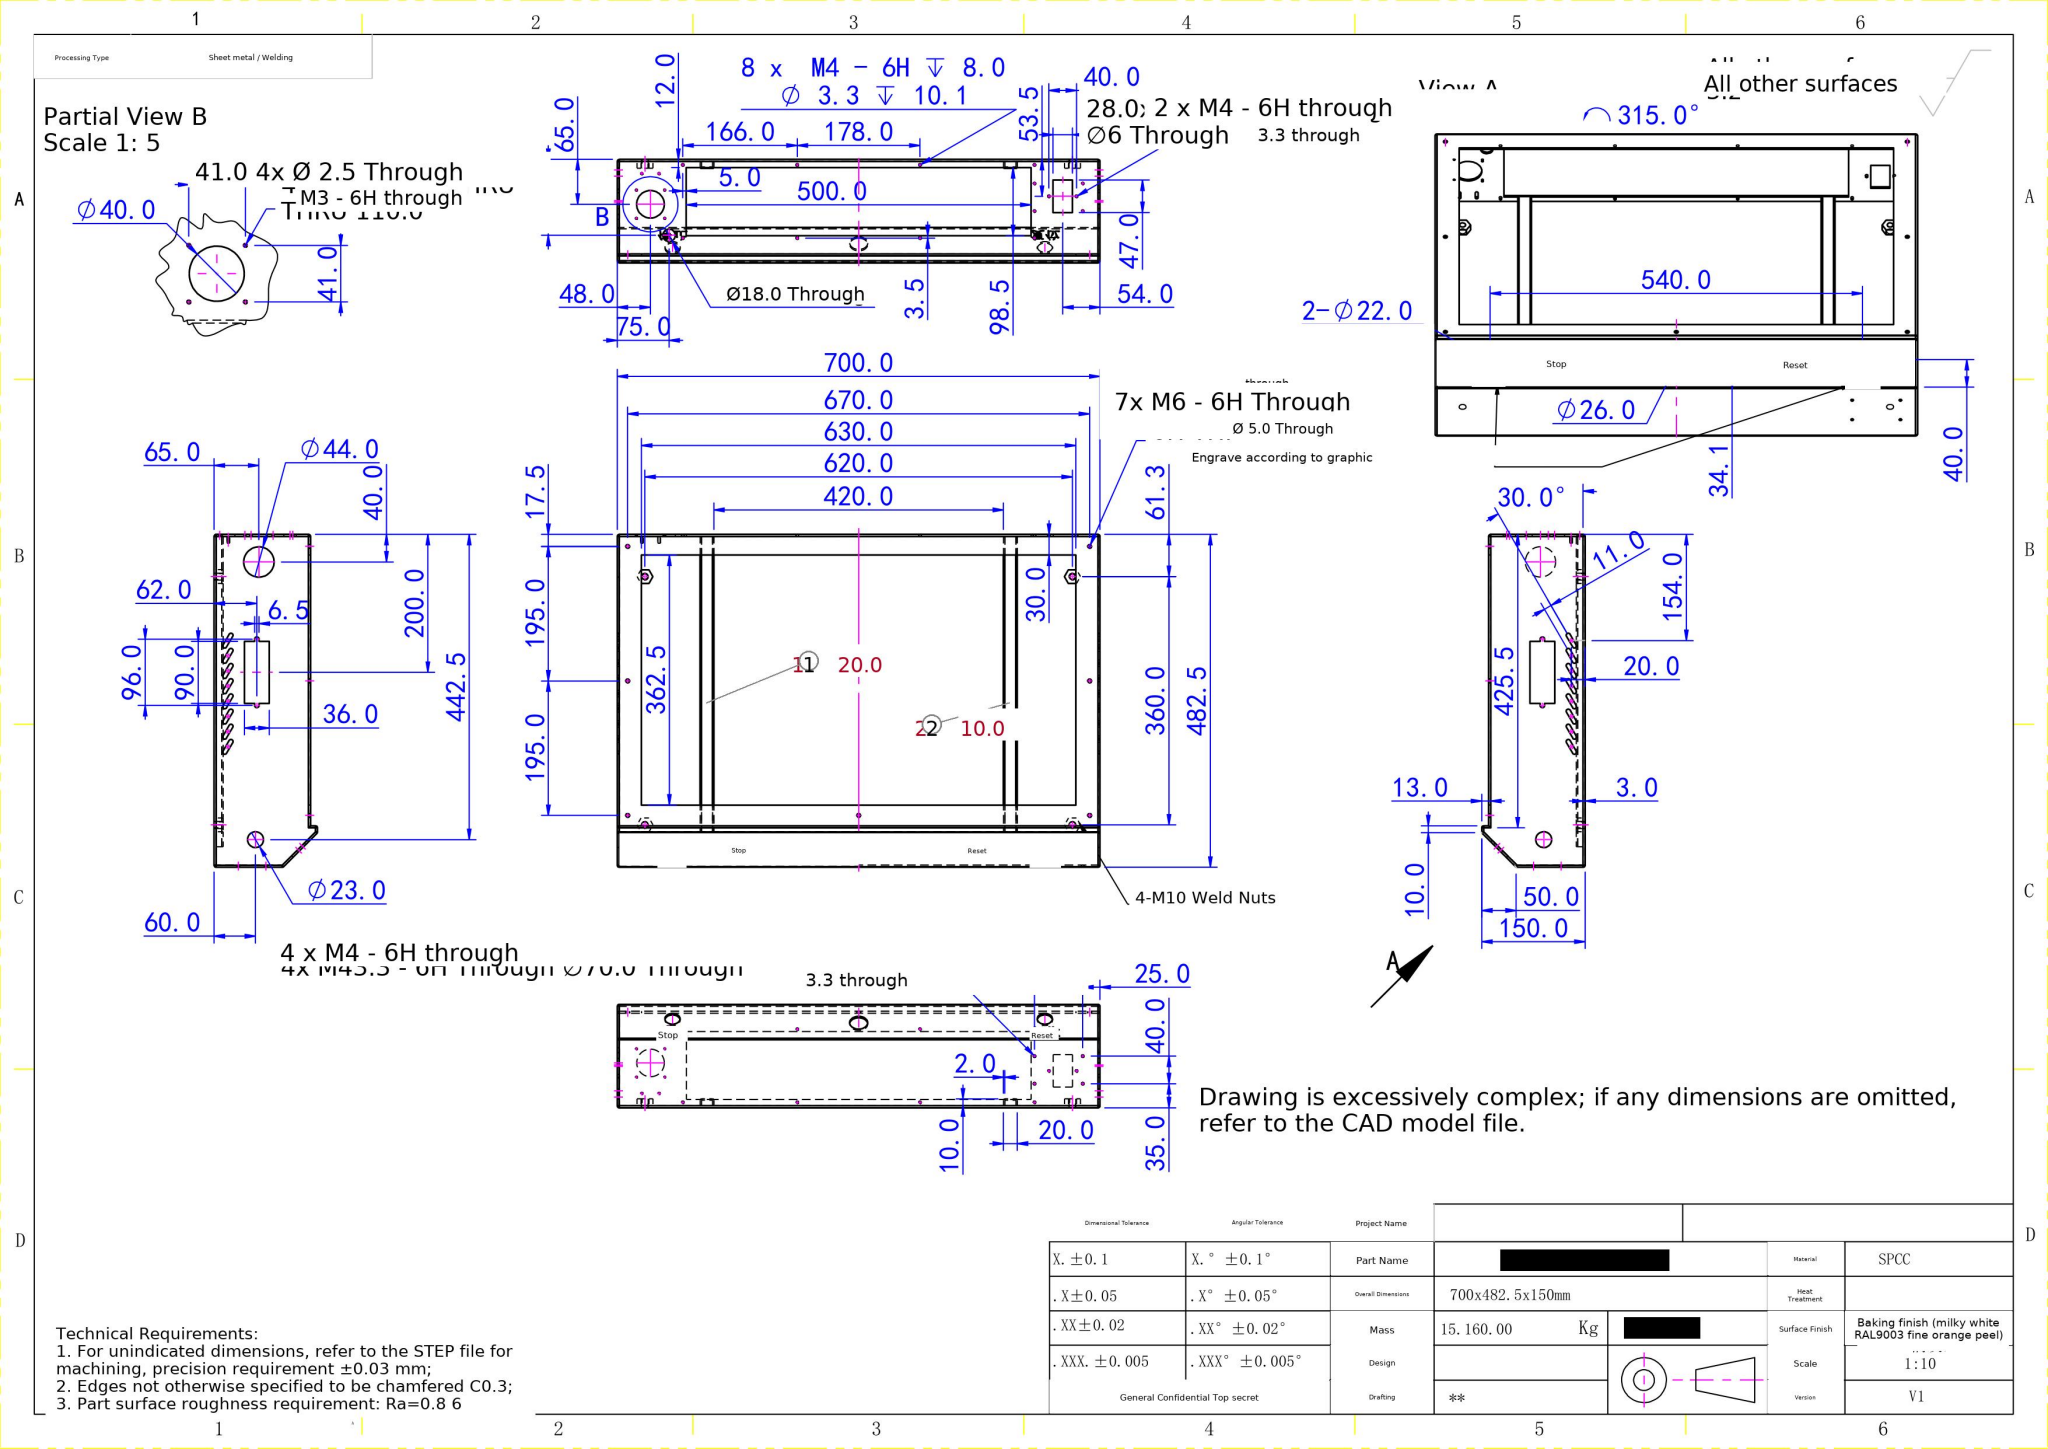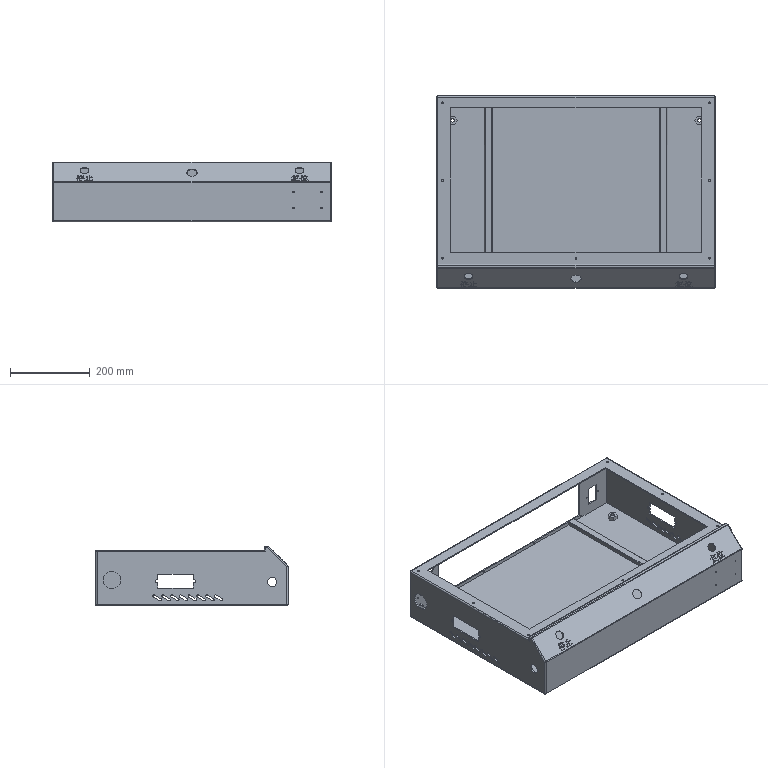Part | SolidWorks | mm | material SPCC | 1 solid | 491 faces | box 700 x 482.5 x 150 mm | volume 2134700 mm3 | plane 271 | cylinder 154 | spline 54 | sphere 12 | commonest cylinder face diameters 6 x68 3.3 x28 5 x14 2.5 x8 4 x8 8.5 x8 23 x4 22 x4